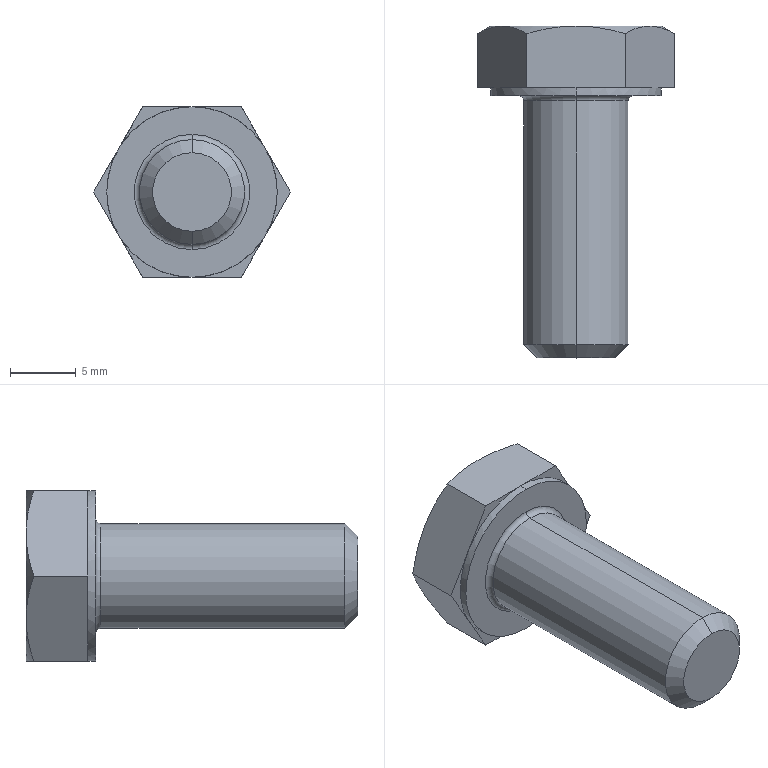Component | SolidWorks | GB_T5781-2000HexHeadBoltFullThreadM8_20-1 | 1 solid | 29 faces | box 15.01 x 25.3 x 13 mm | volume 1760 mm3 | plane 15 | cone 8 | cylinder 4 | torus 2 | commonest cylinder face diameters 8 x2 13 x2 | material 8.8 Grade
build123d program:
from build123d import *

# Parameters (mm, degrees)
BASE_EXTRUDE_DEPTH = 5.3
SKETCH4_W          = 0.6
SKETCH4_H          = 11.006
CHAMFER_2_SIZE     = 1
FILLET_2_R         = 0.4


with BuildPart() as part:
    # Sketch1 → Base-Extrude (new body)
    with BuildSketch(Plane(origin=(0, 0, 0), x_dir=(0, 0, -1), z_dir=(1, 0, 0))):
        Polygon((6.5, 3.753), (6.5, -3.753), (0, -7.506), (-6.5, -3.753), (-6.5, 3.753), (0, 7.506), align=None)
    extrude(amount=BASE_EXTRUDE_DEPTH)

    # Sketch2 → Revolve1 (revolve)
    with BuildSketch(Plane.XY, mode=Mode.PRIVATE) as revolve1_sk:
        Polygon((0, 0), (25.3, 0), (25.3, 2.917), (25.3, 4), (0, 4), align=None)
    revolve(revolve1_sk.sketch.rotate(Axis((0, 0, 0), (1, 0, 0)), 90), axis=Axis((0, 0, 0), (1, 0, 0)))

    # Sketch3 → Cut-Revolve1 (revolve, cut)
    with BuildSketch(Plane.XY):
        Polygon((0, 6.5), (3.467, 12.506), (3.467, 17.506), (-10, 17.506), (-10, 6.5), align=None)
    revolve(axis=Axis((0, 0, 0), (1, 0, 0)), mode=Mode.SUBTRACT)

    # Sketch5 → Cut-Revolve2 (revolve, cut)
    with BuildSketch(Plane.XY):
        Polygon((5.3, 6.5), (1.833, 12.506), (1.833, 17.506), (11.833, 17.506), (11.833, 6.5), align=None)
    revolve(axis=Axis((0, 0, 0), (1, 0, 0)), mode=Mode.SUBTRACT)

    # Sketch4 → Cut-Revolve3 (revolve, cut)
    with BuildSketch(Plane.XY, mode=Mode.PRIVATE) as cut_revolve3_sk:
        with Locations((5, 12.003)):
            Rectangle(SKETCH4_W, SKETCH4_H)
    revolve(cut_revolve3_sk.sketch.rotate(Axis((0, 0, 0), (1, 0, 0)), 270), axis=Axis((0, 0, 0), (1, 0, 0)), mode=Mode.SUBTRACT)

    # Chamfer 2
    chamfer_2_edges = [part.edges().sort_by_distance(p)[0] for p in [
        (25.3, 0, -4),
    ]]
    chamfer(chamfer_2_edges, length=CHAMFER_2_SIZE)

    # Fillet 2
    fillet_2_edges = [part.edges().sort_by_distance(p)[0] for p in [
        (5.3, 0, -4),
    ]]
    fillet(fillet_2_edges, radius=FILLET_2_R)


solid = part.part

# Placed as in the assembly
solid = solid.moved(Location((-40.006, 43, 26), (0, 0, -90)))
STEP:
#1=COLOUR_RGB('',0.7922,0.8196,0.9333);
#2=FILL_AREA_STYLE_COLOUR('',#1);
#3=FILL_AREA_STYLE('',(#2));
#4=SURFACE_STYLE_FILL_AREA(#3);
#5=SURFACE_SIDE_STYLE('',(#4));
#6=SURFACE_STYLE_USAGE(.BOTH.,#5);
#7=PRESENTATION_STYLE_ASSIGNMENT((#6));
#8=CARTESIAN_POINT('',(-1.575,1.469,1.181));
#9=VERTEX_POINT('',#8);
#10=CARTESIAN_POINT('',(-1.575,1.469,0.8661));
#11=VERTEX_POINT('',#10);
#12=CARTESIAN_POINT('',(-1.575,1.469,1.024));
#13=DIRECTION('',(0.,-1.,0.));
#14=DIRECTION('',(0.,0.,-1.));
#15=AXIS2_PLACEMENT_3D('',#12,#13,#14);
#16=CIRCLE('',#15,0.1575);
#17=EDGE_CURVE('',#9,#11,#16,.T.);
#18=ORIENTED_EDGE('',*,*,#17,.F.);
#19=CARTESIAN_POINT('',(-1.575,1.484,1.197));
#20=VERTEX_POINT('',#19);
#21=CARTESIAN_POINT('',(-1.575,1.469,1.197));
#22=DIRECTION('',(1.,0.,-0.));
#23=DIRECTION('',(0.,0.,-1.));
#24=AXIS2_PLACEMENT_3D('',#21,#22,#23);
#25=CIRCLE('',#24,0.01575);
#26=EDGE_CURVE('',#9,#20,#25,.T.);
#27=ORIENTED_EDGE('',*,*,#26,.T.);
#28=CARTESIAN_POINT('',(-1.575,1.484,0.8504));
#29=VERTEX_POINT('',#28);
#30=CARTESIAN_POINT('',(-1.575,1.484,1.024));
#31=DIRECTION('',(0.,1.,0.));
#32=DIRECTION('',(0.,0.,-1.));
#33=AXIS2_PLACEMENT_3D('',#30,#31,#32);
#34=CIRCLE('',#33,0.1732);
#35=EDGE_CURVE('',#29,#20,#34,.T.);
#36=ORIENTED_EDGE('',*,*,#35,.F.);
#37=CARTESIAN_POINT('',(-1.575,1.469,0.8504));
#38=DIRECTION('',(-1.,0.,0.));
#39=DIRECTION('',(0.,0.,1.));
#40=AXIS2_PLACEMENT_3D('',#37,#38,#39);
#41=CIRCLE('',#40,0.01575);
#42=EDGE_CURVE('',#11,#29,#41,.T.);
#43=ORIENTED_EDGE('',*,*,#42,.F.);
#44=EDGE_LOOP('',(#18,#27,#36,#43));
#45=FACE_OUTER_BOUND('',#44,.T.);
#46=CARTESIAN_POINT('',(-1.575,1.469,1.024));
#47=DIRECTION('',(0.,-1.,0.));
#48=DIRECTION('',(0.,0.,-1.));
#49=AXIS2_PLACEMENT_3D('',#46,#47,#48);
#50=TOROIDAL_SURFACE('',#49,0.1732,0.01575);
#51=ADVANCED_FACE('',(#45),#50,.F.);
#52=CARTESIAN_POINT('',(-1.575,0.6969,0.9055));
#53=VERTEX_POINT('',#52);
#54=CARTESIAN_POINT('',(-1.575,0.6969,1.142));
#55=VERTEX_POINT('',#54);
#56=CARTESIAN_POINT('',(-1.575,0.6969,1.024));
#57=DIRECTION('',(0.,-1.,0.));
#58=DIRECTION('',(0.,0.,1.));
#59=AXIS2_PLACEMENT_3D('',#56,#57,#58);
#60=CIRCLE('',#59,0.1181);
#61=EDGE_CURVE('',#53,#55,#60,.T.);
#62=ORIENTED_EDGE('',*,*,#61,.F.);
#63=CARTESIAN_POINT('',(-1.575,0.7362,0.8661));
#64=VERTEX_POINT('',#63);
#65=CARTESIAN_POINT('',(-1.575,0.7362,0.8661));
#66=DIRECTION('',(0.,0.7071,-0.7071));
#67=VECTOR('',#66,39.37);
#68=LINE('',#65,#67);
#69=EDGE_CURVE('',#53,#64,#68,.T.);
#70=ORIENTED_EDGE('',*,*,#69,.T.);
#71=CARTESIAN_POINT('',(-1.575,0.7362,1.181));
#72=VERTEX_POINT('',#71);
#73=CARTESIAN_POINT('',(-1.575,0.7362,1.024));
#74=DIRECTION('',(0.,1.,0.));
#75=DIRECTION('',(0.,0.,1.));
#76=AXIS2_PLACEMENT_3D('',#73,#74,#75);
#77=CIRCLE('',#76,0.1575);
#78=EDGE_CURVE('',#72,#64,#77,.T.);
#79=ORIENTED_EDGE('',*,*,#78,.F.);
#80=CARTESIAN_POINT('',(-1.575,0.7362,1.181));
#81=DIRECTION('',(0.,0.7071,0.7071));
#82=VECTOR('',#81,39.37);
#83=LINE('',#80,#82);
#84=EDGE_CURVE('',#55,#72,#83,.T.);
#85=ORIENTED_EDGE('',*,*,#84,.F.);
#86=EDGE_LOOP('',(#62,#70,#79,#85));
#87=FACE_OUTER_BOUND('',#86,.T.);
#88=CARTESIAN_POINT('',(-1.575,0.7362,1.024));
#89=DIRECTION('',(0.,1.,0.));
#90=DIRECTION('',(0.,0.,1.));
#91=AXIS2_PLACEMENT_3D('',#88,#89,#90);
#92=CONICAL_SURFACE('',#91,0.1575,0.7854);
#93=ADVANCED_FACE('',(#87),#92,.T.);
#94=ORIENTED_EDGE('',*,*,#78,.T.);
#95=CARTESIAN_POINT('',(-1.575,1.693,0.8661));
#96=DIRECTION('',(0.,1.,0.));
#97=VECTOR('',#96,39.37);
#98=LINE('',#95,#97);
#99=EDGE_CURVE('',#64,#11,#98,.T.);
#100=ORIENTED_EDGE('',*,*,#99,.T.);
#101=CARTESIAN_POINT('',(-1.575,1.469,1.024));
#102=DIRECTION('',(0.,-1.,0.));
#103=DIRECTION('',(0.,0.,-1.));
#104=AXIS2_PLACEMENT_3D('',#101,#102,#103);
#105=CIRCLE('',#104,0.1575);
#106=EDGE_CURVE('',#11,#9,#105,.T.);
#107=ORIENTED_EDGE('',*,*,#106,.T.);
#108=CARTESIAN_POINT('',(-1.575,1.693,1.181));
#109=DIRECTION('',(0.,1.,0.));
#110=VECTOR('',#109,39.37);
#111=LINE('',#108,#110);
#112=EDGE_CURVE('',#72,#9,#111,.T.);
#113=ORIENTED_EDGE('',*,*,#112,.F.);
#114=EDGE_LOOP('',(#94,#100,#107,#113));
#115=FACE_OUTER_BOUND('',#114,.T.);
#116=CARTESIAN_POINT('',(-1.575,1.693,1.024));
#117=DIRECTION('',(0.,1.,0.));
#118=DIRECTION('',(0.,0.,1.));
#119=AXIS2_PLACEMENT_3D('',#116,#117,#118);
#120=CYLINDRICAL_SURFACE('',#119,0.1575);
#121=ADVANCED_FACE('',(#115),#120,.T.);
#122=CARTESIAN_POINT('',(-1.575,1.484,0.7677));
#123=VERTEX_POINT('',#122);
#124=CARTESIAN_POINT('',(-1.575,1.484,1.28));
#125=VERTEX_POINT('',#124);
#126=CARTESIAN_POINT('',(-1.575,1.484,1.024));
#127=DIRECTION('',(0.,-1.,0.));
#128=DIRECTION('',(0.,0.,-1.));
#129=AXIS2_PLACEMENT_3D('',#126,#127,#128);
#130=CIRCLE('',#129,0.2559);
#131=EDGE_CURVE('',#123,#125,#130,.T.);
#132=ORIENTED_EDGE('',*,*,#131,.F.);
#133=CARTESIAN_POINT('',(-1.575,1.508,0.7677));
#134=VERTEX_POINT('',#133);
#135=CARTESIAN_POINT('',(-1.575,1.693,0.7677));
#136=DIRECTION('',(0.,1.,0.));
#137=VECTOR('',#136,39.37);
#138=LINE('',#135,#137);
#139=EDGE_CURVE('',#123,#134,#138,.T.);
#140=ORIENTED_EDGE('',*,*,#139,.T.);
#141=CARTESIAN_POINT('',(-1.353,1.508,0.8957));
#142=VERTEX_POINT('',#141);
#143=CARTESIAN_POINT('',(-1.575,1.508,1.024));
#144=DIRECTION('',(0.,1.,0.));
#145=DIRECTION('',(0.,0.,1.));
#146=AXIS2_PLACEMENT_3D('',#143,#144,#145);
#147=CIRCLE('',#146,0.2559);
#148=EDGE_CURVE('',#142,#134,#147,.T.);
#149=ORIENTED_EDGE('',*,*,#148,.F.);
#150=CARTESIAN_POINT('',(-1.353,1.508,1.152));
#151=VERTEX_POINT('',#150);
#152=CARTESIAN_POINT('',(-1.575,1.508,1.024));
#153=DIRECTION('',(0.,1.,0.));
#154=DIRECTION('',(0.,0.,1.));
#155=AXIS2_PLACEMENT_3D('',#152,#153,#154);
#156=CIRCLE('',#155,0.2559);
#157=EDGE_CURVE('',#151,#142,#156,.T.);
#158=ORIENTED_EDGE('',*,*,#157,.F.);
#159=CARTESIAN_POINT('',(-1.575,1.508,1.28));
#160=VERTEX_POINT('',#159);
#161=CARTESIAN_POINT('',(-1.575,1.508,1.024));
#162=DIRECTION('',(0.,1.,0.));
#163=DIRECTION('',(0.,0.,1.));
#164=AXIS2_PLACEMENT_3D('',#161,#162,#163);
#165=CIRCLE('',#164,0.2559);
#166=EDGE_CURVE('',#160,#151,#165,.T.);
#167=ORIENTED_EDGE('',*,*,#166,.F.);
#168=CARTESIAN_POINT('',(-1.575,1.693,1.28));
#169=DIRECTION('',(0.,1.,0.));
#170=VECTOR('',#169,39.37);
#171=LINE('',#168,#170);
#172=EDGE_CURVE('',#125,#160,#171,.T.);
#173=ORIENTED_EDGE('',*,*,#172,.F.);
#174=EDGE_LOOP('',(#132,#140,#149,#158,#167,#173));
#175=FACE_OUTER_BOUND('',#174,.T.);
#176=CARTESIAN_POINT('',(-1.575,1.693,1.024));
#177=DIRECTION('',(0.,1.,0.));
#178=DIRECTION('',(0.,0.,1.));
#179=AXIS2_PLACEMENT_3D('',#176,#177,#178);
#180=CYLINDRICAL_SURFACE('',#179,0.2559);
#181=ADVANCED_FACE('',(#175),#180,.T.);
#182=CARTESIAN_POINT('',(-1.427,1.508,0.7677));
#183=VERTEX_POINT('',#182);
#184=CARTESIAN_POINT('',(-1.427,1.508,0.7677));
#185=DIRECTION('',(0.5,0.,0.866));
#186=VECTOR('',#185,39.37);
#187=LINE('',#184,#186);
#188=EDGE_CURVE('',#183,#142,#187,.T.);
#189=ORIENTED_EDGE('',*,*,#188,.F.);
#190=CARTESIAN_POINT('',(-1.427,1.67,0.7677));
#191=VERTEX_POINT('',#190);
#192=CARTESIAN_POINT('',(-1.427,1.484,0.7677));
#193=DIRECTION('',(0.,1.,0.));
#194=VECTOR('',#193,39.37);
#195=LINE('',#192,#194);
#196=EDGE_CURVE('',#183,#191,#195,.T.);
#197=ORIENTED_EDGE('',*,*,#196,.T.);
#198=CARTESIAN_POINT('',(-1.353,1.693,0.8957));
#199=VERTEX_POINT('',#198);
#200=CARTESIAN_POINT('',(-1.353,1.693,0.8957));
#201=CARTESIAN_POINT('',(-1.36,1.693,0.8848));
#202=CARTESIAN_POINT('',(-1.366,1.692,0.8739));
#203=CARTESIAN_POINT('',(-1.378,1.69,0.8523));
#204=CARTESIAN_POINT('',(-1.385,1.689,0.8416));
#205=CARTESIAN_POINT('',(-1.403,1.683,0.8096));
#206=CARTESIAN_POINT('',(-1.415,1.677,0.7886));
#207=CARTESIAN_POINT('',(-1.427,1.67,0.7677));
#208=B_SPLINE_CURVE_WITH_KNOTS('',3,(#200,#201,#202,#203,#204,#205,#206,#207),.UNSPECIFIED.,.F.,.F.,(4,2,2,4),(0.003797,0.004743,0.005689,0.00758),.UNSPECIFIED.);
#209=EDGE_CURVE('',#199,#191,#208,.T.);
#210=ORIENTED_EDGE('',*,*,#209,.F.);
#211=CARTESIAN_POINT('',(-1.28,1.67,1.024));
#212=VERTEX_POINT('',#211);
#213=CARTESIAN_POINT('',(-1.28,1.67,1.024));
#214=CARTESIAN_POINT('',(-1.292,1.677,1.003));
#215=CARTESIAN_POINT('',(-1.304,1.683,0.9816));
#216=CARTESIAN_POINT('',(-1.328,1.691,0.939));
#217=CARTESIAN_POINT('',(-1.341,1.693,0.9175));
#218=CARTESIAN_POINT('',(-1.353,1.693,0.8957));
#219=B_SPLINE_CURVE_WITH_KNOTS('',3,(#213,#214,#215,#216,#217,#218),.UNSPECIFIED.,.F.,.F.,(4,2,4),(0.00000024,0.001899,0.003797),.UNSPECIFIED.);
#220=EDGE_CURVE('',#212,#199,#219,.T.);
#221=ORIENTED_EDGE('',*,*,#220,.F.);
#222=CARTESIAN_POINT('',(-1.28,1.508,1.024));
#223=VERTEX_POINT('',#222);
#224=CARTESIAN_POINT('',(-1.28,1.484,1.024));
#225=DIRECTION('',(0.,1.,0.));
#226=VECTOR('',#225,39.37);
#227=LINE('',#224,#226);
#228=EDGE_CURVE('',#223,#212,#227,.T.);
#229=ORIENTED_EDGE('',*,*,#228,.F.);
#230=CARTESIAN_POINT('',(-1.427,1.508,0.7677));
#231=DIRECTION('',(0.5,0.,0.866));
#232=VECTOR('',#231,39.37);
#233=LINE('',#230,#232);
#234=EDGE_CURVE('',#142,#223,#233,.T.);
#235=ORIENTED_EDGE('',*,*,#234,.F.);
#236=EDGE_LOOP('',(#189,#197,#210,#221,#229,#235));
#237=FACE_OUTER_BOUND('',#236,.T.);
#238=CARTESIAN_POINT('',(-1.427,1.484,0.7677));
#239=DIRECTION('',(-0.866,0.,0.5));
#240=DIRECTION('',(-0.5,0.,-0.866));
#241=AXIS2_PLACEMENT_3D('',#238,#239,#240);
#242=PLANE('',#241);
#243=ADVANCED_FACE('',(#237),#242,.F.);
#244=CARTESIAN_POINT('',(-1.28,1.508,1.024));
#245=DIRECTION('',(-0.5,0.,0.866));
#246=VECTOR('',#245,39.37);
#247=LINE('',#244,#246);
#248=EDGE_CURVE('',#223,#151,#247,.T.);
#249=ORIENTED_EDGE('',*,*,#248,.F.);
#250=ORIENTED_EDGE('',*,*,#228,.T.);
#251=CARTESIAN_POINT('',(-1.353,1.693,1.152));
#252=VERTEX_POINT('',#251);
#253=CARTESIAN_POINT('',(-1.353,1.693,1.152));
#254=CARTESIAN_POINT('',(-1.347,1.693,1.141));
#255=CARTESIAN_POINT('',(-1.341,1.692,1.13));
#256=CARTESIAN_POINT('',(-1.328,1.69,1.108));
#257=CARTESIAN_POINT('',(-1.322,1.689,1.098));
#258=CARTESIAN_POINT('',(-1.304,1.683,1.066));
#259=CARTESIAN_POINT('',(-1.292,1.677,1.045));
#260=CARTESIAN_POINT('',(-1.28,1.67,1.024));
#261=B_SPLINE_CURVE_WITH_KNOTS('',3,(#253,#254,#255,#256,#257,#258,#259,#260),.UNSPECIFIED.,.F.,.F.,(4,2,2,4),(0.003797,0.004743,0.005689,0.00758),.UNSPECIFIED.);
#262=EDGE_CURVE('',#252,#212,#261,.T.);
#263=ORIENTED_EDGE('',*,*,#262,.F.);
#264=CARTESIAN_POINT('',(-1.427,1.67,1.28));
#265=VERTEX_POINT('',#264);
#266=CARTESIAN_POINT('',(-1.427,1.67,1.28));
#267=CARTESIAN_POINT('',(-1.415,1.677,1.259));
#268=CARTESIAN_POINT('',(-1.403,1.683,1.238));
#269=CARTESIAN_POINT('',(-1.378,1.691,1.195));
#270=CARTESIAN_POINT('',(-1.366,1.693,1.173));
#271=CARTESIAN_POINT('',(-1.353,1.693,1.152));
#272=B_SPLINE_CURVE_WITH_KNOTS('',3,(#266,#267,#268,#269,#270,#271),.UNSPECIFIED.,.F.,.F.,(4,2,4),(0.00000024,0.001899,0.003797),.UNSPECIFIED.);
#273=EDGE_CURVE('',#265,#252,#272,.T.);
#274=ORIENTED_EDGE('',*,*,#273,.F.);
#275=CARTESIAN_POINT('',(-1.427,1.508,1.28));
#276=VERTEX_POINT('',#275);
#277=CARTESIAN_POINT('',(-1.427,1.484,1.28));
#278=DIRECTION('',(0.,1.,0.));
#279=VECTOR('',#278,39.37);
#280=LINE('',#277,#279);
#281=EDGE_CURVE('',#276,#265,#280,.T.);
#282=ORIENTED_EDGE('',*,*,#281,.F.);
#283=CARTESIAN_POINT('',(-1.28,1.508,1.024));
#284=DIRECTION('',(-0.5,0.,0.866));
#285=VECTOR('',#284,39.37);
#286=LINE('',#283,#285);
#287=EDGE_CURVE('',#151,#276,#286,.T.);
#288=ORIENTED_EDGE('',*,*,#287,.F.);
#289=EDGE_LOOP('',(#249,#250,#263,#274,#282,#288));
#290=FACE_OUTER_BOUND('',#289,.T.);
#291=CARTESIAN_POINT('',(-1.28,1.484,1.024));
#292=DIRECTION('',(-0.866,0.,-0.5));
#293=DIRECTION('',(0.5,0.,-0.866));
#294=AXIS2_PLACEMENT_3D('',#291,#292,#293);
#295=PLANE('',#294);
#296=ADVANCED_FACE('',(#290),#295,.F.);
#297=CARTESIAN_POINT('',(-1.427,1.508,1.28));
#298=DIRECTION('',(-1.,0.,0.));
#299=VECTOR('',#298,39.37);
#300=LINE('',#297,#299);
#301=EDGE_CURVE('',#276,#160,#300,.T.);
#302=ORIENTED_EDGE('',*,*,#301,.F.);
#303=ORIENTED_EDGE('',*,*,#281,.T.);
#304=CARTESIAN_POINT('',(-1.575,1.693,1.28));
#305=VERTEX_POINT('',#304);
#306=CARTESIAN_POINT('',(-1.575,1.693,1.28));
#307=CARTESIAN_POINT('',(-1.55,1.693,1.28));
#308=CARTESIAN_POINT('',(-1.525,1.691,1.28));
#309=CARTESIAN_POINT('',(-1.475,1.683,1.28));
#310=CARTESIAN_POINT('',(-1.451,1.677,1.28));
#311=CARTESIAN_POINT('',(-1.427,1.67,1.28));
#312=B_SPLINE_CURVE_WITH_KNOTS('',3,(#306,#307,#308,#309,#310,#311),.UNSPECIFIED.,.F.,.F.,(4,2,4),(0.01067,0.01257,0.01447),.UNSPECIFIED.);
#313=EDGE_CURVE('',#305,#265,#312,.T.);
#314=ORIENTED_EDGE('',*,*,#313,.F.);
#315=CARTESIAN_POINT('',(-1.723,1.67,1.28));
#316=VERTEX_POINT('',#315);
#317=CARTESIAN_POINT('',(-1.723,1.67,1.28));
#318=CARTESIAN_POINT('',(-1.699,1.677,1.28));
#319=CARTESIAN_POINT('',(-1.674,1.683,1.28));
#320=CARTESIAN_POINT('',(-1.625,1.691,1.28));
#321=CARTESIAN_POINT('',(-1.6,1.693,1.28));
#322=CARTESIAN_POINT('',(-1.575,1.693,1.28));
#323=B_SPLINE_CURVE_WITH_KNOTS('',3,(#317,#318,#319,#320,#321,#322),.UNSPECIFIED.,.F.,.F.,(4,2,4),(0.006874,0.008773,0.01067),.UNSPECIFIED.);
#324=EDGE_CURVE('',#316,#305,#323,.T.);
#325=ORIENTED_EDGE('',*,*,#324,.F.);
#326=CARTESIAN_POINT('',(-1.723,1.508,1.28));
#327=VERTEX_POINT('',#326);
#328=CARTESIAN_POINT('',(-1.723,1.484,1.28));
#329=DIRECTION('',(0.,1.,0.));
#330=VECTOR('',#329,39.37);
#331=LINE('',#328,#330);
#332=EDGE_CURVE('',#327,#316,#331,.T.);
#333=ORIENTED_EDGE('',*,*,#332,.F.);
#334=CARTESIAN_POINT('',(-1.427,1.508,1.28));
#335=DIRECTION('',(-1.,0.,0.));
#336=VECTOR('',#335,39.37);
#337=LINE('',#334,#336);
#338=EDGE_CURVE('',#160,#327,#337,.T.);
#339=ORIENTED_EDGE('',*,*,#338,.F.);
#340=EDGE_LOOP('',(#302,#303,#314,#325,#333,#339));
#341=FACE_OUTER_BOUND('',#340,.T.);
#342=CARTESIAN_POINT('',(-1.427,1.484,1.28));
#343=DIRECTION('',(0.,0.,-1.));
#344=DIRECTION('',(0.,1.,0.));
#345=AXIS2_PLACEMENT_3D('',#342,#343,#344);
#346=PLANE('',#345);
#347=ADVANCED_FACE('',(#341),#346,.F.);
#348=CARTESIAN_POINT('',(-1.797,1.508,1.152));
#349=VERTEX_POINT('',#348);
#350=CARTESIAN_POINT('',(-1.871,1.508,1.024));
#351=DIRECTION('',(-0.5,0.,-0.866));
#352=VECTOR('',#351,39.37);
#353=LINE('',#350,#352);
#354=EDGE_CURVE('',#327,#349,#353,.T.);
#355=ORIENTED_EDGE('',*,*,#354,.F.);
#356=ORIENTED_EDGE('',*,*,#332,.T.);
#357=CARTESIAN_POINT('',(-1.797,1.693,1.152));
#358=VERTEX_POINT('',#357);
#359=CARTESIAN_POINT('',(-1.797,1.693,1.152));
#360=CARTESIAN_POINT('',(-1.79,1.693,1.162));
#361=CARTESIAN_POINT('',(-1.784,1.692,1.173));
#362=CARTESIAN_POINT('',(-1.772,1.69,1.195));
#363=CARTESIAN_POINT('',(-1.765,1.689,1.206));
#364=CARTESIAN_POINT('',(-1.747,1.683,1.238));
#365=CARTESIAN_POINT('',(-1.735,1.677,1.259));
#366=CARTESIAN_POINT('',(-1.723,1.67,1.28));
#367=B_SPLINE_CURVE_WITH_KNOTS('',3,(#359,#360,#361,#362,#363,#364,#365,#366),.UNSPECIFIED.,.F.,.F.,(4,2,2,4),(0.003797,0.004743,0.005689,0.00758),.UNSPECIFIED.);
#368=EDGE_CURVE('',#358,#316,#367,.T.);
#369=ORIENTED_EDGE('',*,*,#368,.F.);
#370=CARTESIAN_POINT('',(-1.871,1.67,1.024));
#371=VERTEX_POINT('',#370);
#372=CARTESIAN_POINT('',(-1.871,1.67,1.024));
#373=CARTESIAN_POINT('',(-1.858,1.677,1.045));
#374=CARTESIAN_POINT('',(-1.846,1.683,1.066));
#375=CARTESIAN_POINT('',(-1.822,1.691,1.108));
#376=CARTESIAN_POINT('',(-1.809,1.693,1.13));
#377=CARTESIAN_POINT('',(-1.797,1.693,1.152));
#378=B_SPLINE_CURVE_WITH_KNOTS('',3,(#372,#373,#374,#375,#376,#377),.UNSPECIFIED.,.F.,.F.,(4,2,4),(0.00000024,0.001899,0.003797),.UNSPECIFIED.);
#379=EDGE_CURVE('',#371,#358,#378,.T.);
#380=ORIENTED_EDGE('',*,*,#379,.F.);
#381=CARTESIAN_POINT('',(-1.871,1.508,1.024));
#382=VERTEX_POINT('',#381);
#383=CARTESIAN_POINT('',(-1.871,1.484,1.024));
#384=DIRECTION('',(0.,1.,0.));
#385=VECTOR('',#384,39.37);
#386=LINE('',#383,#385);
#387=EDGE_CURVE('',#382,#371,#386,.T.);
#388=ORIENTED_EDGE('',*,*,#387,.F.);
#389=CARTESIAN_POINT('',(-1.871,1.508,1.024));
#390=DIRECTION('',(-0.5,0.,-0.866));
#391=VECTOR('',#390,39.37);
#392=LINE('',#389,#391);
#393=EDGE_CURVE('',#349,#382,#392,.T.);
#394=ORIENTED_EDGE('',*,*,#393,.F.);
#395=EDGE_LOOP('',(#355,#356,#369,#380,#388,#394));
#396=FACE_OUTER_BOUND('',#395,.T.);
#397=CARTESIAN_POINT('',(-1.871,1.484,1.024));
#398=DIRECTION('',(0.866,0.,-0.5));
#399=DIRECTION('',(0.5,0.,0.866));
#400=AXIS2_PLACEMENT_3D('',#397,#398,#399);
#401=PLANE('',#400);
#402=ADVANCED_FACE('',(#396),#401,.F.);
#403=CARTESIAN_POINT('',(-1.797,1.508,0.8957));
#404=VERTEX_POINT('',#403);
#405=CARTESIAN_POINT('',(-1.723,1.508,0.7677));
#406=DIRECTION('',(0.5,0.,-0.866));
#407=VECTOR('',#406,39.37);
#408=LINE('',#405,#407);
#409=EDGE_CURVE('',#382,#404,#408,.T.);
#410=ORIENTED_EDGE('',*,*,#409,.F.);
#411=ORIENTED_EDGE('',*,*,#387,.T.);
#412=CARTESIAN_POINT('',(-1.797,1.693,0.8957));
#413=VERTEX_POINT('',#412);
#414=CARTESIAN_POINT('',(-1.797,1.693,0.8957));
#415=CARTESIAN_POINT('',(-1.803,1.693,0.9065));
#416=CARTESIAN_POINT('',(-1.809,1.692,0.9174));
#417=CARTESIAN_POINT('',(-1.822,1.69,0.939));
#418=CARTESIAN_POINT('',(-1.828,1.689,0.9497));
#419=CARTESIAN_POINT('',(-1.846,1.683,0.9817));
#420=CARTESIAN_POINT('',(-1.858,1.677,1.003));
#421=CARTESIAN_POINT('',(-1.871,1.67,1.024));
#422=B_SPLINE_CURVE_WITH_KNOTS('',3,(#414,#415,#416,#417,#418,#419,#420,#421),.UNSPECIFIED.,.F.,.F.,(4,2,2,4),(0.003797,0.004743,0.005689,0.00758),.UNSPECIFIED.);
#423=EDGE_CURVE('',#413,#371,#422,.T.);
#424=ORIENTED_EDGE('',*,*,#423,.F.);
#425=CARTESIAN_POINT('',(-1.723,1.67,0.7677));
#426=VERTEX_POINT('',#425);
#427=CARTESIAN_POINT('',(-1.723,1.67,0.7677));
#428=CARTESIAN_POINT('',(-1.735,1.677,0.7886));
#429=CARTESIAN_POINT('',(-1.747,1.683,0.8097));
#430=CARTESIAN_POINT('',(-1.772,1.691,0.8523));
#431=CARTESIAN_POINT('',(-1.784,1.693,0.8739));
#432=CARTESIAN_POINT('',(-1.797,1.693,0.8957));
#433=B_SPLINE_CURVE_WITH_KNOTS('',3,(#427,#428,#429,#430,#431,#432),.UNSPECIFIED.,.F.,.F.,(4,2,4),(0.00000024,0.001899,0.003797),.UNSPECIFIED.);
#434=EDGE_CURVE('',#426,#413,#433,.T.);
#435=ORIENTED_EDGE('',*,*,#434,.F.);
#436=CARTESIAN_POINT('',(-1.723,1.508,0.7677));
#437=VERTEX_POINT('',#436);
#438=CARTESIAN_POINT('',(-1.723,1.484,0.7677));
#439=DIRECTION('',(0.,1.,0.));
#440=VECTOR('',#439,39.37);
#441=LINE('',#438,#440);
#442=EDGE_CURVE('',#437,#426,#441,.T.);
#443=ORIENTED_EDGE('',*,*,#442,.F.);
#444=CARTESIAN_POINT('',(-1.723,1.508,0.7677));
#445=DIRECTION('',(0.5,0.,-0.866));
#446=VECTOR('',#445,39.37);
#447=LINE('',#444,#446);
#448=EDGE_CURVE('',#404,#437,#447,.T.);
#449=ORIENTED_EDGE('',*,*,#448,.F.);
#450=EDGE_LOOP('',(#410,#411,#424,#435,#443,#449));
#451=FACE_OUTER_BOUND('',#450,.T.);
#452=CARTESIAN_POINT('',(-1.723,1.484,0.7677));
#453=DIRECTION('',(0.866,0.,0.5));
#454=DIRECTION('',(-0.5,0.,0.866));
#455=AXIS2_PLACEMENT_3D('',#452,#453,#454);
#456=PLANE('',#455);
#457=ADVANCED_FACE('',(#451),#456,.F.);
#458=CARTESIAN_POINT('',(-1.427,1.508,0.7677));
#459=DIRECTION('',(1.,0.,0.));
#460=VECTOR('',#459,39.37);
#461=LINE('',#458,#460);
#462=EDGE_CURVE('',#437,#134,#461,.T.);
#463=ORIENTED_EDGE('',*,*,#462,.F.);
#464=ORIENTED_EDGE('',*,*,#442,.T.);
#465=CARTESIAN_POINT('',(-1.575,1.693,0.7677));
#466=VERTEX_POINT('',#465);
#467=CARTESIAN_POINT('',(-1.575,1.693,0.7677));
#468=CARTESIAN_POINT('',(-1.6,1.693,0.7677));
#469=CARTESIAN_POINT('',(-1.625,1.691,0.7677));
#470=CARTESIAN_POINT('',(-1.674,1.683,0.7677));
#471=CARTESIAN_POINT('',(-1.699,1.677,0.7677));
#472=CARTESIAN_POINT('',(-1.723,1.67,0.7677));
#473=B_SPLINE_CURVE_WITH_KNOTS('',3,(#467,#468,#469,#470,#471,#472),.UNSPECIFIED.,.F.,.F.,(4,2,4),(0.02294,0.02484,0.02674),.UNSPECIFIED.);
#474=EDGE_CURVE('',#466,#426,#473,.T.);
#475=ORIENTED_EDGE('',*,*,#474,.F.);
#476=CARTESIAN_POINT('',(-1.427,1.67,0.7677));
#477=CARTESIAN_POINT('',(-1.451,1.677,0.7677));
#478=CARTESIAN_POINT('',(-1.475,1.683,0.7677));
#479=CARTESIAN_POINT('',(-1.525,1.691,0.7677));
#480=CARTESIAN_POINT('',(-1.55,1.693,0.7677));
#481=CARTESIAN_POINT('',(-1.575,1.693,0.7677));
#482=B_SPLINE_CURVE_WITH_KNOTS('',3,(#476,#477,#478,#479,#480,#481),.UNSPECIFIED.,.F.,.F.,(4,2,4),(0.01914,0.02104,0.02294),.UNSPECIFIED.);
#483=EDGE_CURVE('',#191,#466,#482,.T.);
#484=ORIENTED_EDGE('',*,*,#483,.F.);
#485=ORIENTED_EDGE('',*,*,#196,.F.);
#486=CARTESIAN_POINT('',(-1.427,1.508,0.7677));
#487=DIRECTION('',(1.,0.,0.));
#488=VECTOR('',#487,39.37);
#489=LINE('',#486,#488);
#490=EDGE_CURVE('',#134,#183,#489,.T.);
#491=ORIENTED_EDGE('',*,*,#490,.F.);
#492=EDGE_LOOP('',(#463,#464,#475,#484,#485,#491));
#493=FACE_OUTER_BOUND('',#492,.T.);
#494=CARTESIAN_POINT('',(-1.427,1.484,0.7677));
#495=DIRECTION('',(-0.,0.,1.));
#496=DIRECTION('',(-1.,0.,-0.));
#497=AXIS2_PLACEMENT_3D('',#494,#495,#496);
#498=PLANE('',#497);
#499=ADVANCED_FACE('',(#493),#498,.F.);
#500=ORIENTED_EDGE('',*,*,#434,.T.);
#501=CARTESIAN_POINT('',(-1.575,1.693,1.024));
#502=DIRECTION('',(0.,-1.,0.));
#503=DIRECTION('',(0.,0.,-1.));
#504=AXIS2_PLACEMENT_3D('',#501,#502,#503);
#505=CIRCLE('',#504,0.2559);
#506=EDGE_CURVE('',#413,#466,#505,.T.);
#507=ORIENTED_EDGE('',*,*,#506,.T.);
#508=ORIENTED_EDGE('',*,*,#474,.T.);
#509=EDGE_LOOP('',(#500,#507,#508));
#510=FACE_OUTER_BOUND('',#509,.T.);
#511=CARTESIAN_POINT('',(-1.575,1.693,1.024));
#512=DIRECTION('',(0.,-1.,0.));
#513=DIRECTION('',(0.,0.,-1.));
#514=AXIS2_PLACEMENT_3D('',#511,#512,#513);
#515=CONICAL_SURFACE('',#514,0.2559,1.047);
#516=ADVANCED_FACE('',(#510),#515,.T.);
#517=ORIENTED_EDGE('',*,*,#379,.T.);
#518=CARTESIAN_POINT('',(-1.575,1.693,1.024));
#519=DIRECTION('',(0.,-1.,0.));
#520=DIRECTION('',(0.,0.,-1.));
#521=AXIS2_PLACEMENT_3D('',#518,#519,#520);
#522=CIRCLE('',#521,0.2559);
#523=EDGE_CURVE('',#358,#413,#522,.T.);
#524=ORIENTED_EDGE('',*,*,#523,.T.);
#525=ORIENTED_EDGE('',*,*,#423,.T.);
#526=EDGE_LOOP('',(#517,#524,#525));
#527=FACE_OUTER_BOUND('',#526,.T.);
#528=CARTESIAN_POINT('',(-1.575,1.693,1.024));
#529=DIRECTION('',(0.,-1.,0.));
#530=DIRECTION('',(0.,0.,-1.));
#531=AXIS2_PLACEMENT_3D('',#528,#529,#530);
#532=CONICAL_SURFACE('',#531,0.2559,1.047);
#533=ADVANCED_FACE('',(#527),#532,.T.);
#534=ORIENTED_EDGE('',*,*,#324,.T.);
#535=CARTESIAN_POINT('',(-1.575,1.693,1.024));
#536=DIRECTION('',(0.,-1.,0.));
#537=DIRECTION('',(0.,0.,-1.));
#538=AXIS2_PLACEMENT_3D('',#535,#536,#537);
#539=CIRCLE('',#538,0.2559);
#540=EDGE_CURVE('',#305,#358,#539,.T.);
#541=ORIENTED_EDGE('',*,*,#540,.T.);
#542=ORIENTED_EDGE('',*,*,#368,.T.);
#543=EDGE_LOOP('',(#534,#541,#542));
#544=FACE_OUTER_BOUND('',#543,.T.);
#545=CARTESIAN_POINT('',(-1.575,1.693,1.024));
#546=DIRECTION('',(0.,-1.,0.));
#547=DIRECTION('',(0.,0.,-1.));
#548=AXIS2_PLACEMENT_3D('',#545,#546,#547);
#549=CONICAL_SURFACE('',#548,0.2559,1.047);
#550=ADVANCED_FACE('',(#544),#549,.T.);
#551=ORIENTED_EDGE('',*,*,#313,.T.);
#552=ORIENTED_EDGE('',*,*,#273,.T.);
#553=CARTESIAN_POINT('',(-1.575,1.693,1.024));
#554=DIRECTION('',(0.,1.,0.));
#555=DIRECTION('',(0.,0.,1.));
#556=AXIS2_PLACEMENT_3D('',#553,#554,#555);
#557=CIRCLE('',#556,0.2559);
#558=EDGE_CURVE('',#305,#252,#557,.T.);
#559=ORIENTED_EDGE('',*,*,#558,.F.);
#560=EDGE_LOOP('',(#551,#552,#559));
#561=FACE_OUTER_BOUND('',#560,.T.);
#562=CARTESIAN_POINT('',(-1.575,1.693,1.024));
#563=DIRECTION('',(0.,-1.,0.));
#564=DIRECTION('',(0.,0.,-1.));
#565=AXIS2_PLACEMENT_3D('',#562,#563,#564);
#566=CONICAL_SURFACE('',#565,0.2559,1.047);
#567=ADVANCED_FACE('',(#561),#566,.T.);
#568=ORIENTED_EDGE('',*,*,#262,.T.);
#569=ORIENTED_EDGE('',*,*,#220,.T.);
#570=CARTESIAN_POINT('',(-1.575,1.693,1.024));
#571=DIRECTION('',(0.,-1.,0.));
#572=DIRECTION('',(0.,0.,-1.));
#573=AXIS2_PLACEMENT_3D('',#570,#571,#572);
#574=CIRCLE('',#573,0.2559);
#575=EDGE_CURVE('',#199,#252,#574,.T.);
#576=ORIENTED_EDGE('',*,*,#575,.T.);
#577=EDGE_LOOP('',(#568,#569,#576));
#578=FACE_OUTER_BOUND('',#577,.T.);
#579=CARTESIAN_POINT('',(-1.575,1.693,1.024));
#580=DIRECTION('',(0.,-1.,0.));
#581=DIRECTION('',(0.,0.,-1.));
#582=AXIS2_PLACEMENT_3D('',#579,#580,#581);
#583=CONICAL_SURFACE('',#582,0.2559,1.047);
#584=ADVANCED_FACE('',(#578),#583,.T.);
#585=ORIENTED_EDGE('',*,*,#209,.T.);
#586=ORIENTED_EDGE('',*,*,#483,.T.);
#587=CARTESIAN_POINT('',(-1.575,1.693,1.024));
#588=DIRECTION('',(0.,-1.,0.));
#589=DIRECTION('',(0.,0.,-1.));
#590=AXIS2_PLACEMENT_3D('',#587,#588,#589);
#591=CIRCLE('',#590,0.2559);
#592=EDGE_CURVE('',#466,#199,#591,.T.);
#593=ORIENTED_EDGE('',*,*,#592,.T.);
#594=EDGE_LOOP('',(#585,#586,#593));
#595=FACE_OUTER_BOUND('',#594,.T.);
#596=CARTESIAN_POINT('',(-1.575,1.693,1.024));
#597=DIRECTION('',(0.,-1.,0.));
#598=DIRECTION('',(0.,0.,-1.));
#599=AXIS2_PLACEMENT_3D('',#596,#597,#598);
#600=CONICAL_SURFACE('',#599,0.2559,1.047);
#601=ADVANCED_FACE('',(#595),#600,.T.);
#602=ORIENTED_EDGE('',*,*,#592,.F.);
#603=ORIENTED_EDGE('',*,*,#506,.F.);
#604=ORIENTED_EDGE('',*,*,#523,.F.);
#605=ORIENTED_EDGE('',*,*,#540,.F.);
#606=ORIENTED_EDGE('',*,*,#558,.T.);
#607=ORIENTED_EDGE('',*,*,#575,.F.);
#608=EDGE_LOOP('',(#602,#603,#604,#605,#606,#607));
#609=FACE_OUTER_BOUND('',#608,.T.);
#610=CARTESIAN_POINT('',(-1.28,1.693,1.024));
#611=DIRECTION('',(0.,-1.,0.));
#612=DIRECTION('',(0.,0.,-1.));
#613=AXIS2_PLACEMENT_3D('',#610,#611,#612);
#614=PLANE('',#613);
#615=ADVANCED_FACE('',(#609),#614,.F.);
#616=ORIENTED_EDGE('',*,*,#188,.T.);
#617=ORIENTED_EDGE('',*,*,#148,.T.);
#618=ORIENTED_EDGE('',*,*,#490,.T.);
#619=EDGE_LOOP('',(#616,#617,#618));
#620=FACE_OUTER_BOUND('',#619,.T.);
#621=CARTESIAN_POINT('',(-1.319,1.508,1.024));
#622=DIRECTION('',(0.,-1.,0.));
#623=DIRECTION('',(0.,0.,-1.));
#624=AXIS2_PLACEMENT_3D('',#621,#622,#623);
#625=PLANE('',#624);
#626=ADVANCED_FACE('',(#620),#625,.T.);
#627=ORIENTED_EDGE('',*,*,#234,.T.);
#628=ORIENTED_EDGE('',*,*,#248,.T.);
#629=ORIENTED_EDGE('',*,*,#157,.T.);
#630=EDGE_LOOP('',(#627,#628,#629));
#631=FACE_OUTER_BOUND('',#630,.T.);
#632=CARTESIAN_POINT('',(-1.319,1.508,1.024));
#633=DIRECTION('',(0.,-1.,0.));
#634=DIRECTION('',(0.,0.,-1.));
#635=AXIS2_PLACEMENT_3D('',#632,#633,#634);
#636=PLANE('',#635);
#637=ADVANCED_FACE('',(#631),#636,.T.);
#638=ORIENTED_EDGE('',*,*,#287,.T.);
#639=ORIENTED_EDGE('',*,*,#301,.T.);
#640=ORIENTED_EDGE('',*,*,#166,.T.);
#641=EDGE_LOOP('',(#638,#639,#640));
#642=FACE_OUTER_BOUND('',#641,.T.);
#643=CARTESIAN_POINT('',(-1.319,1.508,1.024));
#644=DIRECTION('',(0.,-1.,0.));
#645=DIRECTION('',(0.,0.,-1.));
#646=AXIS2_PLACEMENT_3D('',#643,#644,#645);
#647=PLANE('',#646);
#648=ADVANCED_FACE('',(#642),#647,.T.);
#649=ORIENTED_EDGE('',*,*,#338,.T.);
#650=ORIENTED_EDGE('',*,*,#354,.T.);
#651=CARTESIAN_POINT('',(-1.575,1.508,1.024));
#652=DIRECTION('',(0.,1.,0.));
#653=DIRECTION('',(0.,0.,1.));
#654=AXIS2_PLACEMENT_3D('',#651,#652,#653);
#655=CIRCLE('',#654,0.2559);
#656=EDGE_CURVE('',#349,#160,#655,.T.);
#657=ORIENTED_EDGE('',*,*,#656,.T.);
#658=EDGE_LOOP('',(#649,#650,#657));
#659=FACE_OUTER_BOUND('',#658,.T.);
#660=CARTESIAN_POINT('',(-1.319,1.508,1.024));
#661=DIRECTION('',(0.,-1.,0.));
#662=DIRECTION('',(0.,0.,-1.));
#663=AXIS2_PLACEMENT_3D('',#660,#661,#662);
#664=PLANE('',#663);
#665=ADVANCED_FACE('',(#659),#664,.T.);
#666=ORIENTED_EDGE('',*,*,#393,.T.);
#667=ORIENTED_EDGE('',*,*,#409,.T.);
#668=CARTESIAN_POINT('',(-1.575,1.508,1.024));
#669=DIRECTION('',(0.,1.,0.));
#670=DIRECTION('',(0.,0.,1.));
#671=AXIS2_PLACEMENT_3D('',#668,#669,#670);
#672=CIRCLE('',#671,0.2559);
#673=EDGE_CURVE('',#404,#349,#672,.T.);
#674=ORIENTED_EDGE('',*,*,#673,.T.);
#675=EDGE_LOOP('',(#666,#667,#674));
#676=FACE_OUTER_BOUND('',#675,.T.);
#677=CARTESIAN_POINT('',(-1.319,1.508,1.024));
#678=DIRECTION('',(0.,-1.,0.));
#679=DIRECTION('',(0.,0.,-1.));
#680=AXIS2_PLACEMENT_3D('',#677,#678,#679);
#681=PLANE('',#680);
#682=ADVANCED_FACE('',(#676),#681,.T.);
#683=ORIENTED_EDGE('',*,*,#448,.T.);
#684=ORIENTED_EDGE('',*,*,#462,.T.);
#685=CARTESIAN_POINT('',(-1.575,1.508,1.024));
#686=DIRECTION('',(0.,1.,0.));
#687=DIRECTION('',(0.,0.,1.));
#688=AXIS2_PLACEMENT_3D('',#685,#686,#687);
#689=CIRCLE('',#688,0.2559);
#690=EDGE_CURVE('',#134,#404,#689,.T.);
#691=ORIENTED_EDGE('',*,*,#690,.T.);
#692=EDGE_LOOP('',(#683,#684,#691));
#693=FACE_OUTER_BOUND('',#692,.T.);
#694=CARTESIAN_POINT('',(-1.319,1.508,1.024));
#695=DIRECTION('',(0.,-1.,0.));
#696=DIRECTION('',(0.,0.,-1.));
#697=AXIS2_PLACEMENT_3D('',#694,#695,#696);
#698=PLANE('',#697);
#699=ADVANCED_FACE('',(#693),#698,.T.);
#700=ORIENTED_EDGE('',*,*,#139,.F.);
#701=CARTESIAN_POINT('',(-1.575,1.484,1.024));
#702=DIRECTION('',(0.,-1.,0.));
#703=DIRECTION('',(0.,0.,-1.));
#704=AXIS2_PLACEMENT_3D('',#701,#702,#703);
#705=CIRCLE('',#704,0.2559);
#706=EDGE_CURVE('',#125,#123,#705,.T.);
#707=ORIENTED_EDGE('',*,*,#706,.F.);
#708=ORIENTED_EDGE('',*,*,#172,.T.);
#709=ORIENTED_EDGE('',*,*,#656,.F.);
#710=ORIENTED_EDGE('',*,*,#673,.F.);
#711=ORIENTED_EDGE('',*,*,#690,.F.);
#712=EDGE_LOOP('',(#700,#707,#708,#709,#710,#711));
#713=FACE_OUTER_BOUND('',#712,.T.);
#714=CARTESIAN_POINT('',(-1.575,1.693,1.024));
#715=DIRECTION('',(0.,1.,0.));
#716=DIRECTION('',(0.,0.,1.));
#717=AXIS2_PLACEMENT_3D('',#714,#715,#716);
#718=CYLINDRICAL_SURFACE('',#717,0.2559);
#719=ADVANCED_FACE('',(#713),#718,.T.);
#720=CARTESIAN_POINT('',(-1.575,0.6969,1.024));
#721=DIRECTION('',(0.,-1.,0.));
#722=DIRECTION('',(0.,0.,1.));
#723=AXIS2_PLACEMENT_3D('',#720,#721,#722);
#724=CIRCLE('',#723,0.1181);
#725=EDGE_CURVE('',#55,#53,#724,.T.);
#726=ORIENTED_EDGE('',*,*,#725,.T.);
#727=ORIENTED_EDGE('',*,*,#61,.T.);
#728=EDGE_LOOP('',(#726,#727));
#729=FACE_OUTER_BOUND('',#728,.T.);
#730=CARTESIAN_POINT('',(-1.575,0.6969,1.024));
#731=DIRECTION('',(0.,1.,0.));
#732=DIRECTION('',(0.,0.,1.));
#733=AXIS2_PLACEMENT_3D('',#730,#731,#732);
#734=PLANE('',#733);
#735=ADVANCED_FACE('',(#729),#734,.F.);
#736=ORIENTED_EDGE('',*,*,#99,.F.);
#737=CARTESIAN_POINT('',(-1.575,0.7362,1.024));
#738=DIRECTION('',(0.,1.,0.));
#739=DIRECTION('',(0.,0.,1.));
#740=AXIS2_PLACEMENT_3D('',#737,#738,#739);
#741=CIRCLE('',#740,0.1575);
#742=EDGE_CURVE('',#64,#72,#741,.T.);
#743=ORIENTED_EDGE('',*,*,#742,.T.);
#744=ORIENTED_EDGE('',*,*,#112,.T.);
#745=ORIENTED_EDGE('',*,*,#17,.T.);
#746=EDGE_LOOP('',(#736,#743,#744,#745));
#747=FACE_OUTER_BOUND('',#746,.T.);
#748=CARTESIAN_POINT('',(-1.575,1.693,1.024));
#749=DIRECTION('',(0.,1.,0.));
#750=DIRECTION('',(0.,0.,1.));
#751=AXIS2_PLACEMENT_3D('',#748,#749,#750);
#752=CYLINDRICAL_SURFACE('',#751,0.1575);
#753=ADVANCED_FACE('',(#747),#752,.T.);
#754=ORIENTED_EDGE('',*,*,#35,.T.);
#755=CARTESIAN_POINT('',(-1.575,1.484,1.024));
#756=DIRECTION('',(0.,1.,0.));
#757=DIRECTION('',(0.,0.,-1.));
#758=AXIS2_PLACEMENT_3D('',#755,#756,#757);
#759=CIRCLE('',#758,0.1732);
#760=EDGE_CURVE('',#20,#29,#759,.T.);
#761=ORIENTED_EDGE('',*,*,#760,.T.);
#762=EDGE_LOOP('',(#754,#761));
#763=FACE_BOUND('',#762,.T.);
#764=ORIENTED_EDGE('',*,*,#706,.T.);
#765=ORIENTED_EDGE('',*,*,#131,.T.);
#766=EDGE_LOOP('',(#764,#765));
#767=FACE_OUTER_BOUND('',#766,.T.);
#768=CARTESIAN_POINT('',(-1.28,1.484,1.024));
#769=DIRECTION('',(0.,-1.,0.));
#770=DIRECTION('',(0.,0.,-1.));
#771=AXIS2_PLACEMENT_3D('',#768,#769,#770);
#772=PLANE('',#771);
#773=ADVANCED_FACE('',(#763,#767),#772,.T.);
#774=ORIENTED_EDGE('',*,*,#69,.F.);
#775=ORIENTED_EDGE('',*,*,#725,.F.);
#776=ORIENTED_EDGE('',*,*,#84,.T.);
#777=ORIENTED_EDGE('',*,*,#742,.F.);
#778=EDGE_LOOP('',(#774,#775,#776,#777));
#779=FACE_OUTER_BOUND('',#778,.T.);
#780=CARTESIAN_POINT('',(-1.575,0.7362,1.024));
#781=DIRECTION('',(0.,1.,0.));
#782=DIRECTION('',(0.,0.,1.));
#783=AXIS2_PLACEMENT_3D('',#780,#781,#782);
#784=CONICAL_SURFACE('',#783,0.1575,0.7854);
#785=ADVANCED_FACE('',(#779),#784,.T.);
#786=ORIENTED_EDGE('',*,*,#26,.F.);
#787=ORIENTED_EDGE('',*,*,#106,.F.);
#788=ORIENTED_EDGE('',*,*,#42,.T.);
#789=ORIENTED_EDGE('',*,*,#760,.F.);
#790=EDGE_LOOP('',(#786,#787,#788,#789));
#791=FACE_OUTER_BOUND('',#790,.T.);
#792=CARTESIAN_POINT('',(-1.575,1.469,1.024));
#793=DIRECTION('',(0.,-1.,0.));
#794=DIRECTION('',(0.,0.,-1.));
#795=AXIS2_PLACEMENT_3D('',#792,#793,#794);
#796=TOROIDAL_SURFACE('',#795,0.1732,0.01575);
#797=ADVANCED_FACE('',(#791),#796,.F.);
#798=CLOSED_SHELL('',(#51,#93,#121,#181,#243,#296,#347,#402,#457,#499,#516,#533,#550,#567,#584,#601,#615,#626,#637,#648,#665,#682,#699,#719,#735,#753,#773,#785,#797));
#799=MANIFOLD_SOLID_BREP('',#798);
#800=STYLED_ITEM('',(#7),#799);
#801=PRESENTATION_LAYER_ASSIGNMENT('','',(#800));
#802=CARTESIAN_POINT('',(0.,0.,0.));
#803=DIRECTION('',(0.,0.,1.));
#804=DIRECTION('',(1.,0.,0.));
#805=AXIS2_PLACEMENT_3D('',#802,#803,#804);
#806=(LENGTH_UNIT()NAMED_UNIT(*)SI_UNIT($,.METRE.));
#807=LENGTH_MEASURE_WITH_UNIT(LENGTH_MEASURE(0.0254),#806);
#808=DIMENSIONAL_EXPONENTS(1.,0.,0.,0.,0.,0.,0.);
#809=(CONVERSION_BASED_UNIT('',#807)LENGTH_UNIT()NAMED_UNIT(#808));
#810=UNCERTAINTY_MEASURE_WITH_UNIT(LENGTH_MEASURE(0.00001),#809,'','');
#811=(NAMED_UNIT(*)PLANE_ANGLE_UNIT()SI_UNIT($,.RADIAN.));
#812=(NAMED_UNIT(*)SI_UNIT($,.STERADIAN.)SOLID_ANGLE_UNIT());
#813=(GEOMETRIC_REPRESENTATION_CONTEXT(3)GLOBAL_UNCERTAINTY_ASSIGNED_CONTEXT((#810))GLOBAL_UNIT_ASSIGNED_CONTEXT((#809,#811,#812))REPRESENTATION_CONTEXT('',''));
#814=ADVANCED_BREP_SHAPE_REPRESENTATION('',(#799,#805),#813);
#815=(LENGTH_UNIT()NAMED_UNIT(*)SI_UNIT($,.METRE.));
#816=LENGTH_MEASURE_WITH_UNIT(LENGTH_MEASURE(0.0254),#815);
#817=DIMENSIONAL_EXPONENTS(1.,0.,0.,0.,0.,0.,0.);
#818=(CONVERSION_BASED_UNIT('',#816)LENGTH_UNIT()NAMED_UNIT(#817));
#819=UNCERTAINTY_MEASURE_WITH_UNIT(LENGTH_MEASURE(0.00001),#818,'','');
#820=(NAMED_UNIT(*)PLANE_ANGLE_UNIT()SI_UNIT($,.RADIAN.));
#821=(NAMED_UNIT(*)SI_UNIT($,.STERADIAN.)SOLID_ANGLE_UNIT());
#822=(GEOMETRIC_REPRESENTATION_CONTEXT(3)GLOBAL_UNCERTAINTY_ASSIGNED_CONTEXT((#819))GLOBAL_UNIT_ASSIGNED_CONTEXT((#818,#820,#821))REPRESENTATION_CONTEXT('',''));
#823=MECHANICAL_DESIGN_GEOMETRIC_PRESENTATION_REPRESENTATION('',(#800),#822);